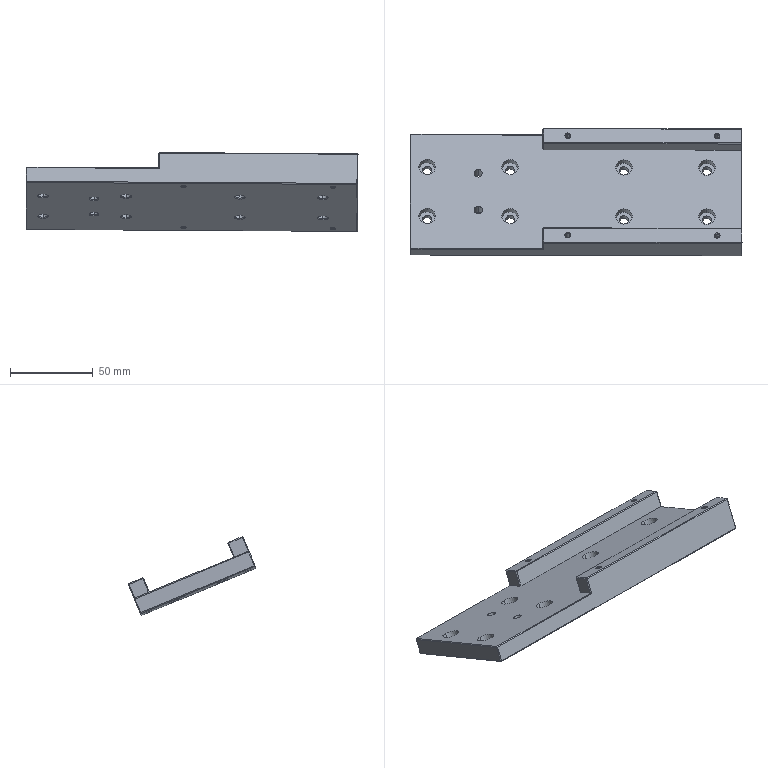Component | SolidWorks | 12-1 | 1 solid | 136 faces | box 200.13 x 76.84 x 47.49 mm | volume 168554 mm3 | cylinder 48 | plane 48 | cone 40 | commonest cylinder face diameters 10 x16 5.5 x16 2.5 x8 5 x4 3.3 x4
build123d program:
from build123d import *

# Parameters (mm, degrees)
SKETCH1_W                                       = 75
SKETCH1_H                                       = 200
BOSS_EXTRUDE1_DEPTH                             = 20
SKETCH2_W                                       = 55
SKETCH2_H                                       = 20
CUT_EXTRUDE1_DEPTH                              = 205.466
SKETCH3_W                                       = 75
SKETCH3_H                                       = 80
CUT_EXTRUDE2_DEPTH                              = 10
M4_TAPPED_HOLE1_D                               = 3.3
M4_TAPPED_HOLE1_DEPTH                           = 10.1
M4_TAPPED_HOLE1_TIP                             = 0.9914
M5_HEX_SOCKET_HEAD_CAP_SCREW_CBORE1_D           = 5.5
M5_HEX_SOCKET_HEAD_CAP_SCREW_CBORE1_CBORE_D     = 10
M5_HEX_SOCKET_HEAD_CAP_SCREW_CBORE1_CBORE_DEPTH = 5.4
LPATTERN1_COUNT                                 = 2
LPATTERN1_PITCH                                 = 50
LPATTERN2_COUNT                                 = 2
LPATTERN2_PITCH                                 = 118.6
LPATTERN2_COPY_1_D                              = 5.5
LPATTERN2_COPY_1_CBORE_D                        = 10
LPATTERN2_COPY_1_CBORE_DEPTH                    = 5.4
M3_TAPPED_HOLE1_D                               = 2.5
M6_TAPPED_HOLE1_D                               = 5
M6_TAPPED_HOLE1_DEPTH                           = 15
M6_TAPPED_HOLE1_TIP                             = 1.502
CHAMFER1_SIZE                                   = 0.5
CHAMFER2_SIZE                                   = 0.5


with BuildPart() as part:
    # Sketch1 → Boss-Extrude1 (new body)
    with BuildSketch(Plane.XY):
        Rectangle(SKETCH1_W, SKETCH1_H)
    extrude(amount=BOSS_EXTRUDE1_DEPTH)

    # Sketch2 → Cut-Extrude1 (cut, through all)
    with BuildSketch(Plane(origin=(0, -100, 0), x_dir=(-1, 0, 0), z_dir=(0, -1, 0))):
        Rectangle(SKETCH2_W, SKETCH2_H)
    extrude(amount=-CUT_EXTRUDE1_DEPTH, mode=Mode.SUBTRACT)

    # Sketch3 → Cut-Extrude2 (cut)
    with BuildSketch(Plane(origin=(0, 0, 0), x_dir=(-1, 0, 0), z_dir=(0, 0, -1))):
        with Locations((0, -60)):
            Rectangle(SKETCH3_W, SKETCH3_H)
    extrude(amount=-CUT_EXTRUDE2_DEPTH, mode=Mode.SUBTRACT)

    # M4 Tapped Hole1
    with Locations(Plane(origin=(37.5, 0, 0), x_dir=(0, 0, -1), z_dir=(1, 0, 0))):
        with Locations((-15, -60), (-15, -70)):
            Hole(M4_TAPPED_HOLE1_D / 2, depth=M4_TAPPED_HOLE1_DEPTH)
            with Locations((0, 0, -(M4_TAPPED_HOLE1_DEPTH + M4_TAPPED_HOLE1_TIP / 2))):  # 118° drill point
                Cone(0, M4_TAPPED_HOLE1_D / 2, M4_TAPPED_HOLE1_TIP, mode=Mode.SUBTRACT)

    # M5 Hex Socket Head Cap Screw CBORE1 (through all)
    with Locations(Plane(origin=(0, 0, 10), x_dir=(-1, 0, 0), z_dir=(0, 0, -1))):
        with Locations((-16, 78.9), (16, 78.9)):
            m5_hex_socket_head_cap_screw_cbore1 = CounterBoreHole(M5_HEX_SOCKET_HEAD_CAP_SCREW_CBORE1_D / 2, M5_HEX_SOCKET_HEAD_CAP_SCREW_CBORE1_CBORE_D / 2, M5_HEX_SOCKET_HEAD_CAP_SCREW_CBORE1_CBORE_DEPTH)

    # LPattern1: M5 Hex Socket Head Cap Screw CBORE1 ×2
    with Locations(*[(0, -i * LPATTERN1_PITCH, 0) for i in range(1, LPATTERN1_COUNT)]):
        add(m5_hex_socket_head_cap_screw_cbore1, mode=Mode.SUBTRACT)

    # LPattern2: M5 Hex Socket Head Cap Screw CBORE1 ×2
    with Locations(*[(0, -i * LPATTERN2_PITCH, 0) for i in range(1, LPATTERN2_COUNT)]):
        add(m5_hex_socket_head_cap_screw_cbore1, mode=Mode.SUBTRACT)

    # LPattern2 copy 1 (through all)
    with Locations(Plane(origin=(0, -168.6, 10), x_dir=(-1, 0, 0), z_dir=(0, 0, -1))):
        with Locations((-16, 78.9), (16, 78.9)):
            CounterBoreHole(LPATTERN2_COPY_1_D / 2, LPATTERN2_COPY_1_CBORE_D / 2, LPATTERN2_COPY_1_CBORE_DEPTH)

    # M3 Tapped Hole1 (through all)
    with Locations(Plane(origin=(0, 0, 0), x_dir=(-1, 0, 0), z_dir=(0, 0, -1))):
        with Locations((32.5, 85), (32.5, -5), (-32.5, -5), (-32.5, 85)):
            Hole(M3_TAPPED_HOLE1_D / 2)

    # M6 Tapped Hole1
    with Locations(Plane(origin=(0, 0, 10), x_dir=(-1, 0, 0), z_dir=(0, 0, -1))):
        with Locations((-12, -59), (12, -59)):
            Hole(M6_TAPPED_HOLE1_D / 2, depth=M6_TAPPED_HOLE1_DEPTH)
            with Locations((0, 0, -(M6_TAPPED_HOLE1_DEPTH + M6_TAPPED_HOLE1_TIP / 2))):  # 118° drill point
                Cone(0, M6_TAPPED_HOLE1_D / 2, M6_TAPPED_HOLE1_TIP, mode=Mode.SUBTRACT)

    # Chamfer1
    chamfer1_edges = [part.edges().sort_by_distance(p)[0] for p in [
        (-37.5, 0, 20),
        (-18.75, -89.7, 20),
        (-18.75, -39.7, 20),
        (13.25, -39.7, 20),
        (13.25, -89.7, 20),
        (31.25, 85, 0),
        (0, -100, 20),
        (31.25, 85, 20),
        (31.25, -5, 0),
        (31.25, -5, 20),
        (-33.75, -5, 0),
        (-33.75, -5, 20),
        (-33.75, 85, 0),
        (-33.75, 85, 20),
        (-32.5, 100, 0),
        (-27.5, 40, 0),
        (-14.5, -59, 20),
        (9.5, -59, 20),
        (27.5, 40, 0),
        (37.5, 40, 0),
        (37.5, 0, 20),
        (32.5, -20, 0),
        (-32.5, -20, 0),
        (-37.5, 40, 0),
        (32.5, 100, 0),
        (0, 100, 20),
        (-18.75, 78.9, 20),
        (13.25, 78.9, 20),
        (13.25, 28.9, 20),
        (-18.75, 28.9, 20),
    ]]
    chamfer(chamfer1_edges, length=CHAMFER1_SIZE)

    # Chamfer2
    chamfer2_edges = [part.edges().sort_by_distance(p)[0] for p in [
        (-37.5, -100, 14.75),
        (37.5, -100, 14.75),
        (-37.5, 100, 10),
        (27.5, 100, 5.25),
        (37.5, 100, 10),
        (-27.5, 100, 5.25),
        (27.5, -20, 5.25),
        (0, -100, 10),
        (0, 100, 10),
        (37.5, -20, 5.25),
        (-27.5, -20, 5.25),
        (37.5, -60, 10),
        (-37.5, -60, 10),
        (-37.5, -20, 5.25),
    ]]
    chamfer(chamfer2_edges, length=CHAMFER2_SIZE)


solid = part.part

# Placed as in the assembly
solid = solid.moved(Location((73.885, -76.038, 450.212), (157.516, -0.3658, -90.008)))